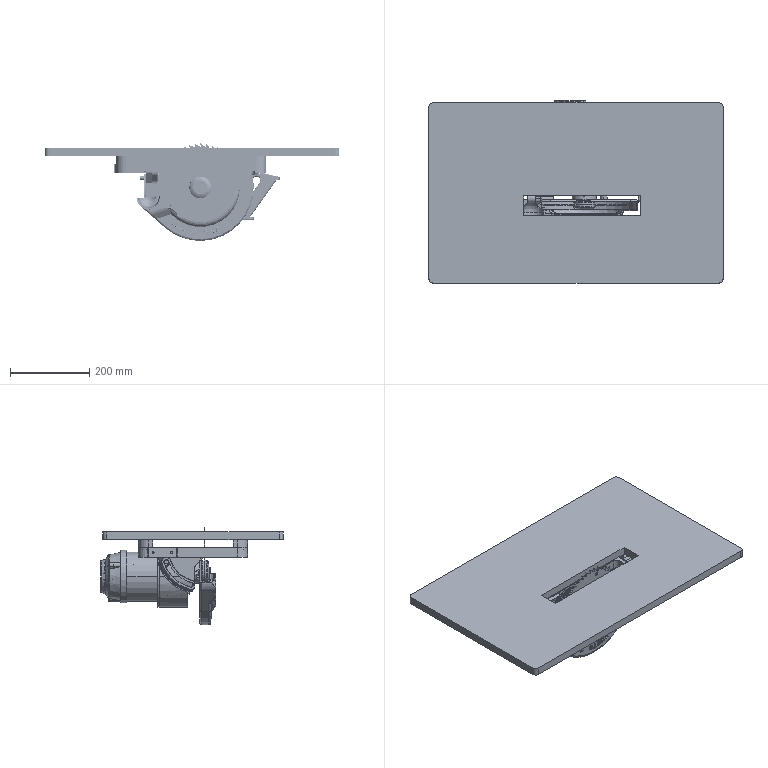Assembly | SolidWorks | mm | 26 component files | 27 solids | 6740 faces | box 740.79 x 458.78 x 246.36 mm | volume 9916213 mm3 | plane 3141 | cylinder 1972 | spline 1003 | torus 509 | cone 89 | sphere 26 | commonest cylinder face diameters 4 x526 6 x152 2 x122 0.4 x100 1.771 x86 1.996 x71 74 x59 1 x52
Bill of materials:
Angle | 1 |  | Quarter-round sector plate with a perpendicular flat top flange, a curved rim along the arc, an arc-shaped through slot, and a small eye lug with a hole and short cylindrical boss at one corner.
Axe | 1 |  | Plain rectangular bar/block, apparently square in cross-section, with flat faces; no holes or features visible.
Base | 1 |  | Thin rectangular plate with slightly rounded corners and a central rectangular through slot, with a frame-like protrusion on the underside around the slot.
Blade cover | 1 |  | Circular disc/washer-like part with a central through hole and a chamfered or domed edge on one face.
Blade holder | 1 |  | Flanged hub: circular flange disc with a central keyed bore, a cylindrical hub on both sides, and two small pins/bosses projecting from one face.
Blade | 1 |  | Thin circular toothed disc that looks like a saw blade, with many angled teeth, a central bore, two small holes near the bore, and four radial slots ending in round holes near the edge.
Bmper fest | 1 |  | Solid plain cylinder with flat ends; no holes, chamfers or other features visible.
Cache cable | 1 |  | Half-cylindrical saddle/clamp half with a semicircular bore that has a central raised band or groove, flat side mounting flanges each with one through hole, and a triangular rib on the outer underside.
cache ein aus | 1 |  | Open hood-like bracket/enclosure with a curved side profile, one open face, a large circular opening with a cylindrical collar on the back, small holes, and a lug with a hole at one corner.
Cache Festo AD85 | 1 |  | Round stepped cup/housing with an outer flange, tapered body, internal cross-shaped spokes holding a central round hub, and three small mounting holes in bosses around the rim.
Circlips | 1 |  | Open split ring of round wire with both ends bent inward toward the center, leaving a gap.
Electrical box | 1 |  | Rectangular block-like housing with rounded edges, a hollow rectangular cavity open at one end, rows of small holes on one face, protruding rounded pins/rails, and a projecting tab with two upright pins on one side.
Engrenange 30 | 1 |  | Spur gear with a long cylindrical shaft sticking out of one face; the shaft has a short keyway or flat-key feature near its free end.
Filtre moteur | 1 |  | Thin flat circular disc cut through with a regular grid of rectangular openings, like a mesh, screen or perforated grille.
Garde scie int | 1 |  | Dark, roughly half-disc (D-shaped) plate. It has a central round through-hole with a raised collar, a curved raised rib inside the edge, a rounded knob or lobe at one corner, and stepped or pointed edge projections along the straight side.
Gear cover festo | 1 |  | Flange plate with an irregular, rounded-triangular outline and a cylindrical hub on one side. The hub has a central through-bore, and there are mounting holes around the flange.
Gear cover | 1 |  | Thin flat annular disc (washer or gasket-like ring) with a large central hole and four small holes evenly spaced on a bolt circle.
Gearbox Housing | 1 |  | Shallow cylindrical cup or drum with a lip at the open rim. The closed end face has a crescent-shaped area of many round perforations, several small holes, a central bore and an internal hub with a lobed opening.
Int_rieur Stator | 1 |  | Cylindrical cage-like assembly or part: a central solid cylindrical sleeve between two rounded end rings, joined by a ring of evenly spaced axial bars. The bore is hollow and the outer flange has arc-shaped slots.
Interrupteur haut | 1 |  | Flat rectangular mounting base with side tabs and a raised half-cylindrical saddle or clamp boss in the middle. The boss has a through-hole along its axis, and the plate has several through-holes.
Pignon 20T | 1 |  | Spur gear with a cylindrical hub on one face and a central bore with a keyway.
Plaque signal_tique Festo | 1 |  | Thin, slightly curved rectangular plate with rounded corners and four small corner holes. One face has raised or engraved text and lines, consistent with a label or nameplate layout.
Poussoir | 1 |  | Lever or handle: a thick circular hub with a square (diamond-oriented) through-hole and a straight rectangular arm extending out to a rounded or chamfered tip.
Rotor | 1 |  | Rotor-like rotating body: a cylindrical core with faint skewed lines on its surface, mounted on a stepped shaft that sticks out from both ends. Each end face carries about six radial fin- or blade-like projections.
Stator | 1 |  | Thin-walled cylindrical sleeve with an outward radial flange near one end and a short stepped spigot past the flange. The flange outline is mostly circular but cut off flat across one side.
Top base | 1 |  | Long, complex frame or housing. One end has a large circular ring opening, and the frame extends lengthwise into an open, angled truss-like arm with rectangular openings and box sections. Several cylindrical pins stick out from the ends.
Mates:
1. concentric | cache ein aus-1 face at (46.207, 122.2, -73.22) dir (0, 0, 1) r 1.5 | Cache cable-1 edge at (46.207, 122.2, -26.555) dir (0, 0, 1) r 2
2. concentric | cache ein aus-1 face at (74.207, 122.2, -73.22) dir (0, 0, 1) r 1.5 | Cache cable-1 face at (74.207, 122.2, -35.055) dir (0, 0, 1) r 2
3. coincident | Base-1 face at (-224.172, -146.57, 1.945) dir (0, 0, -1) | Angle-1 face at (-113.172, 78.95, 1.945) dir (0, 0, 1)
4. concentric | Base-1 edge at (-124.172, 46.93, 1.945) dir (0, 0, 1) r 3.15 | Angle-1 face at (-124.172, 46.93, -98.751) dir (0, 0, 1) r 3
5. concentric | Base-1 face at (-124.172, 6.93, 1.945) dir (0, 0, 1) r 3.15 | Angle-1 face at (-124.172, 6.93, -98.751) dir (0, 0, 1) r 3
6. concentric | Angle-1 face at (-113.172, -23.8, 1.945) dir (-1, 0, 0) r 4 | Top base-1 face at (-146.172, -23.8, 1.945) dir (1, 0, 0) r 4
7. concentric | Gearbox Housing-1 face at (-46.672, 54.2, -61.055) dir (0, -1, 0) r 65 | Top base-1 face at (-46.672, 76.201, -61.055) dir (0, -1, 0) r 65
8. coincident | Gearbox Housing-1 edge at (-46.672, 4.2, -61.055) dir (0, 1, 0) r 62 | Top base-1 face at (128.328, 4.2, 7.945) dir (0, -1, 0)
9. coincident | Base-1 face at (135.828, -10.07, 11.945) dir (-1, 0, 0) | Top base-1 face at (135.828, 76.2, 7.945) dir (1, 0, 0)
10. coincident | cache ein aus-1 face at (-6.64, 111.2, 7.945) dir (0, 0, 1) | Top base-1 face at (188.328, -33.8, 7.945) dir (0, 0, 1)
11. coincident | cache ein aus-1 face at (115.165, 111.2, 7.945) dir (1, 0, 0) | Top base-1 face at (115.165, 56.2, -21.349) dir (1, 0, 0)
12. coincident | cache ein aus-1 face at (-6.64, 111.2, 7.945) dir (0, 0, 1) | Top base-1 face at (188.328, -33.8, 7.945) dir (0, 0, 1)
13. coincident | cache ein aus-1 face at (46.207, 136.2, -17.055) dir (0, 0, -1) | Cache cable-1 face at (42.207, 136.95, -17.055) dir (0, 0, 1)
14. coincident | cache ein aus-1 face at (-6.64, 111.2, 7.945) dir (0, 0, 1) | Top base-1 face at (188.328, -33.8, 7.945) dir (0, 0, 1)
15. coincident | cache ein aus-1 face at (115.165, 111.2, 7.945) dir (1, 0, 0) | Top base-1 face at (115.165, 56.2, -21.349) dir (1, 0, 0)
16. coincident | cache ein aus-1 face at (-6.64, 76.2, 7.945) dir (0, -1, 0) | Top base-1 face at (188.328, 76.2, -139.055) dir (0, 1, 0)
17. concentric | Gearbox Housing-1 face at (-46.672, 4.2, -61.055) dir (0, 1, 0) r 9 | Rotor-1 face at (-46.672, 7.2, -61.055) dir (0, 1, 0) r 8
18. distance | Rotor-1 face at (-46.672, 51.075, -61.055) dir (-0.4731, 0, 0.881) r 1.875 | Gearbox Housing-1 face at (-46.672, 48.2, -61.055) dir (0, 1, 0)
19. concentric | Rotor-1 face at (-46.672, 7.2, -61.055) dir (0, 1, 0) r 8 | Pignon 20T-1 face at (-46.672, 8.2, -61.055) dir (0, 1, 0) r 8
20. coincident | Rotor-1 face at (-37.678, 14.2, -58.779) dir (0.881, 0, 0.4731) | Pignon 20T-1 face at (-38.743, 8.2, -56.797) dir (-0.881, 0, -0.4731)
21. coincident | Gearbox Housing-1 face at (-46.672, 29.2, -61.055) dir (0, -1, 0) | Pignon 20T-1 face at (-46.672, 29.2, -61.055) dir (0, 1, 0)
22. coincident | Top base-1 face at (-46.672, 75.2, -61.055) dir (0, 1, 0) | Stator-1 face at (-46.672, 75.2, -61.055) dir (0, -1, 0)
23. concentric | Top base-1 face at (-46.672, -33.801, -133.055) dir (0, 1, 0) r 2 | Stator-1 face at (-46.672, 160.201, -133.055) dir (0, -1, 0) r 2.75
24. concentric | Cache Festo AD85-2/Cache Festo AD85-1 face at (-46.672, -499842.3, -118.055) dir (0, 1, 0) r 2.685 | Stator-1 face at (-46.672, 140.2, -118.055) dir (0, 1, 0) r 2.2
25. coincident | Cache Festo AD85-2/Cache Festo AD85-1 face at (13.328, 157.7, -61.055) dir (0, -1, 0) | Stator-1 face at (-46.672, 157.7, -61.055) dir (0, 1, 0)
26. concentric | Top base-1 face at (-46.672, 76.2, -61.055) dir (0, -1, 0) r 78 | Stator-1 face at (-46.672, 160.2, -61.055) dir (0, -1, 0) r 78
27. concentric | Cache Festo AD85-2/Cache Festo AD85-1 face at (-46.672, 157.7, -61.055) dir (0, -1, 0) r 66.25 | Stator-1 face at (-46.672, 80.2, -61.055) dir (0, 1, 0) r 62
28. concentric | Stator-1 face at (-46.672, 160.2, -61.055) dir (0, -1, 0) r 58.5 | Int_rieur Stator-1 face at (-46.672, 44.2, -61.055) dir (0, 1, 0) r 58.5
29. coincident | Stator-1 edge at (2.692, 145.2, -32.555) dir (0, 1, 0) r 4 | Int_rieur Stator-1 face at (-46.672, 145.2, -61.055) dir (0, 1, 0)
30. parallel | Top base-1 face at (188.328, 76.2, -129.055) dir (0, 0, -1) | Stator-1 plane at (-46.672, 63.2, -61.055) dir (0, 0, -1)
31. perpendicular | Top base-1 face at (188.328, 76.2, -129.055) dir (0, 0, -1) | Int_rieur Stator-1 plane at (-46.672, 106.7, -61.055) dir (1, 0, 0)
32. coincident | Axe-1 face at (66.718, 84.7, -43.569) dir (-0.7356, 0, 0.6774) | Poussoir-1 face at (66.718, 75.2, -43.569) dir (0.7356, 0, -0.6774)
33. coincident | Axe-1 face at (64.686, 84.7, -45.775) dir (-0.6774, 0, -0.7356) | Poussoir-1 face at (64.686, 75.2, -45.775) dir (0.6774, 0, 0.7356)
34. distance | Axe-1 face at (66.806, 57.7, -45.688) dir (0, -1, 0) | Poussoir-1 face at (66.806, 67.2, -45.688) dir (0, -1, 0)
35. concentric | Interrupteur haut-1 face at (66.806, 100.211, -45.688) dir (0, -1, 0) r 8.755 | Poussoir-1 face at (66.806, 75.2, -45.688) dir (0, -1, 0) r 8.625
36. distance | Axe-1 face at (66.806, 84.7, -45.688) dir (0, 1, 0) | Interrupteur haut-1 face at (55.975, 80.7, -49.833) dir (0, 1, 0)
37. coincident | Electrical box-1 face at (67.484, 71.2, -46.921) dir (0.4823, 0, -0.876) | Interrupteur haut-1 face at (92.232, 51.2, -33.297) dir (-0.4823, 0, 0.876)
38. coincident | Electrical box-1 face at (46.241, 79.7, -58.616) dir (-0.876, 0, -0.4823) | Interrupteur haut-1 face at (47.929, 91.2, -61.682) dir (-0.876, 0, -0.4823)
39. coincident | Electrical box-1 face at (88.728, 51.2, -35.226) dir (0, -1, 0) | Interrupteur haut-1 face at (47.929, 51.2, -61.682) dir (0, -1, 0)
40. concentric | Top base-1 face at (-28.824, 71.2, 81.36) dir (0.4823, 0, -0.876) r 1.75 | Interrupteur haut-1 face at (49.462, 71.2, -60.838) dir (-0.4823, 0, 0.876) r 1.6
41. concentric | Top base-1 face at (10.597, 71.2, 103.062) dir (0.4823, 0, -0.876) r 1.75 | Interrupteur haut-1 face at (88.883, 71.2, -39.136) dir (-0.4823, 0, 0.876) r 1.6
42. coincident | Top base-1 edge at (94.577, 76.2, -36.001) dir (-0.876, 0, -0.4823) | Interrupteur haut-1 face at (93.92, 51.2, -36.363) dir (0.4823, 0, -0.876)
43. coincident | Gearbox Housing-1 face at (-46.672, 4.2, -61.055) dir (0, -1, 0) | Gear cover festo-1 face at (-46.672, 4.2, -61.055) dir (0, 1, 0)
44. concentric | Gearbox Housing-1 face at (-37.987, 58.2, -84.498) dir (0, -1, 0) r 2 | Gear cover festo-1 face at (-37.987, -3.8, -84.498) dir (0, 1, 0) r 2.7
45. concentric | Gearbox Housing-1 face at (-70.115, 58.2, -69.74) dir (0, -1, 0) r 2 | Gear cover festo-1 face at (-70.115, -3.8, -69.74) dir (0, 1, 0) r 2.7
46. concentric | Gear cover festo-1 face at (-11.038, -3.8, -47.854) dir (0, 1, 0) r 8.5 | Engrenange 30-1 face at (-11.038, -41.8, -47.854) dir (0, 1, 0) r 8.5
47. coincident | Pignon 20T-1 face at (-46.672, 8.2, -61.055) dir (0, -1, 0) | Engrenange 30-1 face at (-11.038, 8.2, -47.854) dir (0, -1, 0)
48. gear | Engrenange 30-1 face at (-11.038, 23.2, -47.854) dir (0, -1, 0) r 24 | Pignon 20T-1 face at (-46.672, 8.2, -61.055) dir (0, 1, 0) r 16.5
49. concentric | Gear cover festo-1 face at (-11.038, -29.3, -47.854) dir (0, 1, 0) r 25 | Garde scie int-1 face at (-11.038, -66.3, -47.854) dir (0, 1, 0) r 25
50. tangent | Top base-1 face at (-123.672, -24.478, -55.322) dir (0, 1, 0) r 5 | Garde scie int-1 face at (-88.398, -18.3, -55.051) dir (-0.1342, 0, -0.991)
51. concentric | Engrenange 30-1 face at (-11.038, -41.8, -47.854) dir (0, 1, 0) r 8.5 | Gear cover-1 face at (-11.038, -30.8, -47.854) dir (0, 1, 0) r 14
52. concentric | Gear cover festo-1 face at (-3.669, -14.3, -67.746) dir (0, -1, 0) r 1.5 | Gear cover-1 face at (-3.669, -30.8, -67.746) dir (0, 1, 0) r 2
53. coincident | Garde scie int-1 face at (-11.038, -29.3, -47.854) dir (0, -1, 0) | Gear cover-1 edge at (-11.038, -29.3, -47.854) dir (0, -1, 0) r 36
54. concentric | Engrenange 30-1 face at (-11.038, -41.8, -47.854) dir (0, 1, 0) r 8.5 | Blade holder-1 face at (-11.038, -42.3, -47.854) dir (0, -1, 0) r 8.5
55. concentric | Engrenange 30-1 face at (-11.038, -41.8, -47.854) dir (0, 1, 0) r 8.5 | Blade holder-1 face at (-11.038, -42.3, -47.854) dir (0, -1, 0) r 8.5
56. parallel | Engrenange 30-1 face at (-13.828, -29.8, -38.085) dir (-0.4585, 0, 0.8887) | Blade holder-1 face at (-17.401, -42.3, -39.884) dir (0.4585, 0, -0.8887)
57. coincident | Gear cover-1 face at (-11.038, -30.8, -47.854) dir (0, -1, 0) | Blade holder-1 face at (12.956, -30.8, -35.475) dir (0, 1, 0)
58. concentric | Blade holder-1 face at (-11.038, -42.3, -47.854) dir (0, -1, 0) r 14.75 | Blade-1 face at (-11.038, -37.3, -47.854) dir (0, -1, 0) r 15
59. concentric | Blade holder-1 edge at (7.624, -39.8, -38.226) dir (0, 1, 0) r 2.5 | Blade-1 face at (7.624, -37.3, -38.226) dir (0, -1, 0) r 3
60. coincident | Blade holder-1 face at (2.07, -37.3, -41.091) dir (0, -1, 0) | Blade-1 face at (-11.038, -37.3, -47.854) dir (0, 1, 0)
61. concentric | Blade holder-1 face at (-11.038, -42.3, -47.854) dir (0, -1, 0) r 14.75 | Blade cover-1 face at (-11.038, -39.3, -47.854) dir (0, 1, 0) r 15
62. coincident | Blade-1 face at (-11.038, -39.3, -47.854) dir (0, -1, 0) | Blade cover-1 face at (12.462, -39.3, -40.928) dir (0, 1, 0)
63. concentric | Garde scie int-1 face at (38.344, -19.3, -30.931) dir (0.03868, 0, -0.9993) r 5 | Bmper fest-1 face at (38.344, -19.3, -30.931) dir (0.03868, 0, -0.9993) r 5
64. coincident | Garde scie int-1 face at (38.344, -19.3, -30.931) dir (0.03868, 0, -0.9993) | Bmper fest-1 face at (38.344, -19.3, -30.931) dir (-0.03868, 0, 0.9993)
65. concentric | Stator-1 face at (-46.672, 80.2, -61.055) dir (0, 1, 0) r 62 | Plaque signal_tique Festo-1 edge at (-46.672, 145.2, -61.055) dir (0, -1, 0) r 62
66. distance | Plaque signal_tique Festo-1 face at (-46.672, 95.2, -61.055) dir (0, -1, 0) | Stator-1 face at (-46.672, 80.2, -61.055) dir (0, 1, 0)
67. angle | Top base-1 face at (188.328, 76.2, -129.055) dir (0, 0, -1) | Plaque signal_tique Festo-1 face at (-29.011, 95.2, -122.138) dir (0.08716, 0, -0.9962)
68. coincident | Cache Festo AD85-2/Cache Festo AD85-1 edge at (-46.672, 217.7, -61.055) dir (0, 1, 0) r 35 | Filtre moteur-1 face at (-46.672, 217.7, -61.055) dir (0, -1, 0)
69. concentric | Cache Festo AD85-2/Cache Festo AD85-1 face at (-46.672, 216.2, -61.055) dir (0, 1, 0) r 5.5 | Filtre moteur-1 face at (-46.672, 218.7, -61.055) dir (0, -1, 0) r 37
70. parallel | Base-1 face at (130.828, 103.43, 7.945) dir (0, 0, -1) | Top base-1 face at (188.328, -33.8, 7.945) dir (0, 0, 1)
71. parallel | Circlips-1 plane at (-50.54, 40.339, 0) dir (0, -1, 0) | Cache Festo AD85 plane at (0, 0, 0) dir (0, 1, 0)
72. tangent | Cache Festo AD85-1 face at (-50.54, -22.661, 0) dir (0, -1, 0) r 38 | Circlips-1 face at (-50.54, 39.339, 0) dir (1, 0, 0)
73. tangent | Cache Festo AD85-1 face at (-12.54, 38.339, 0) dir (0, 1, 0) | Circlips-1 face at (-50.54, 39.339, 0) dir (1, 0, 0)